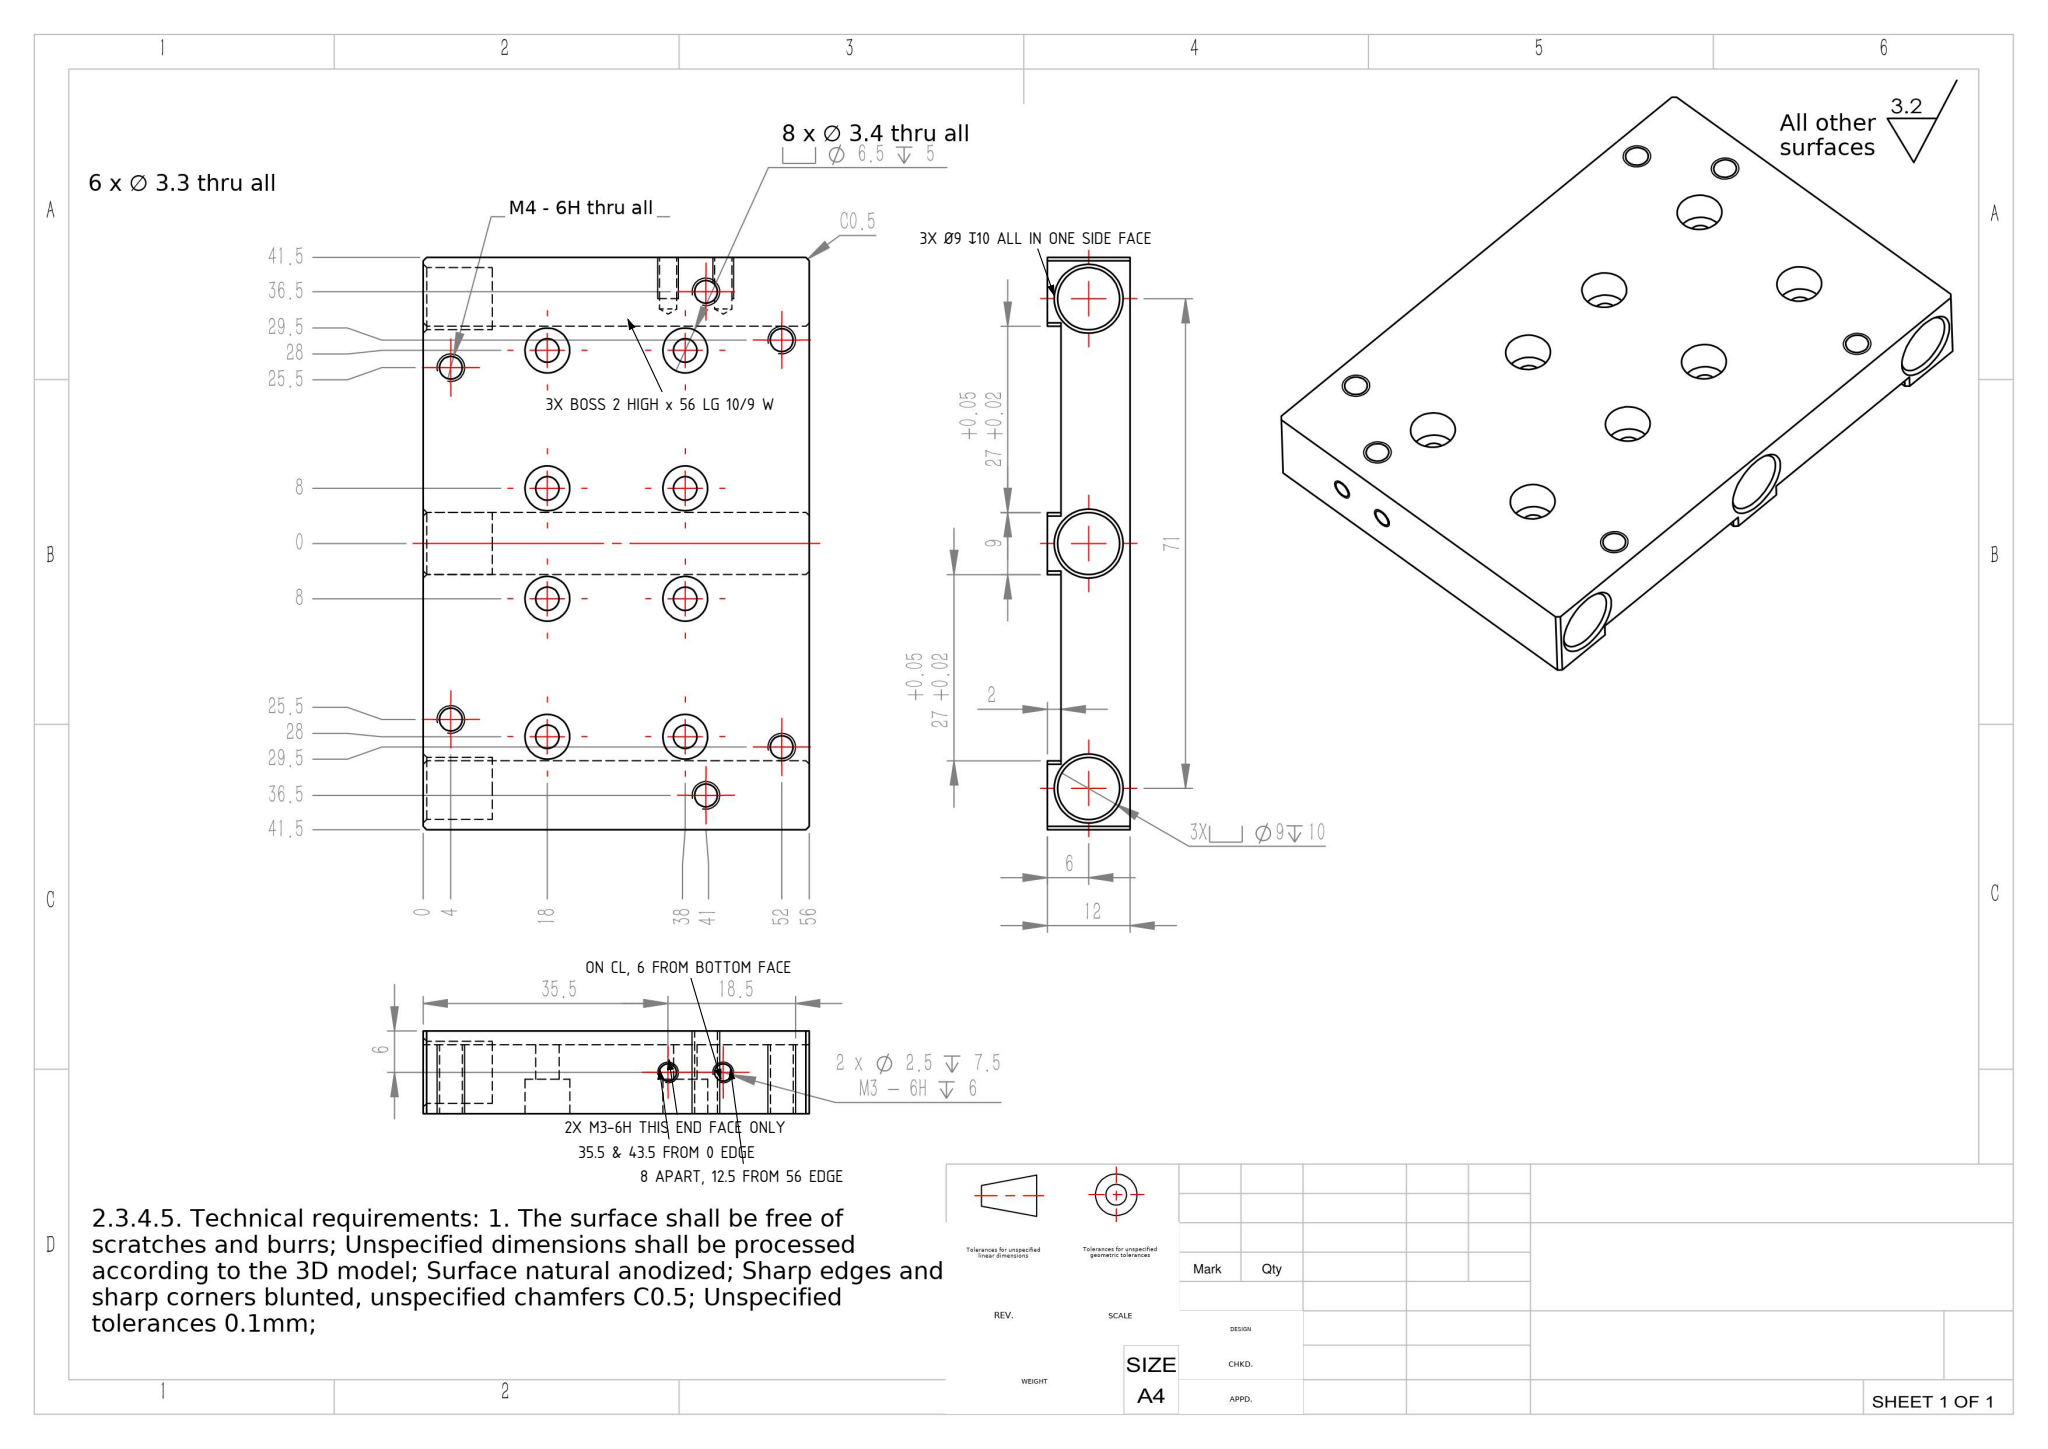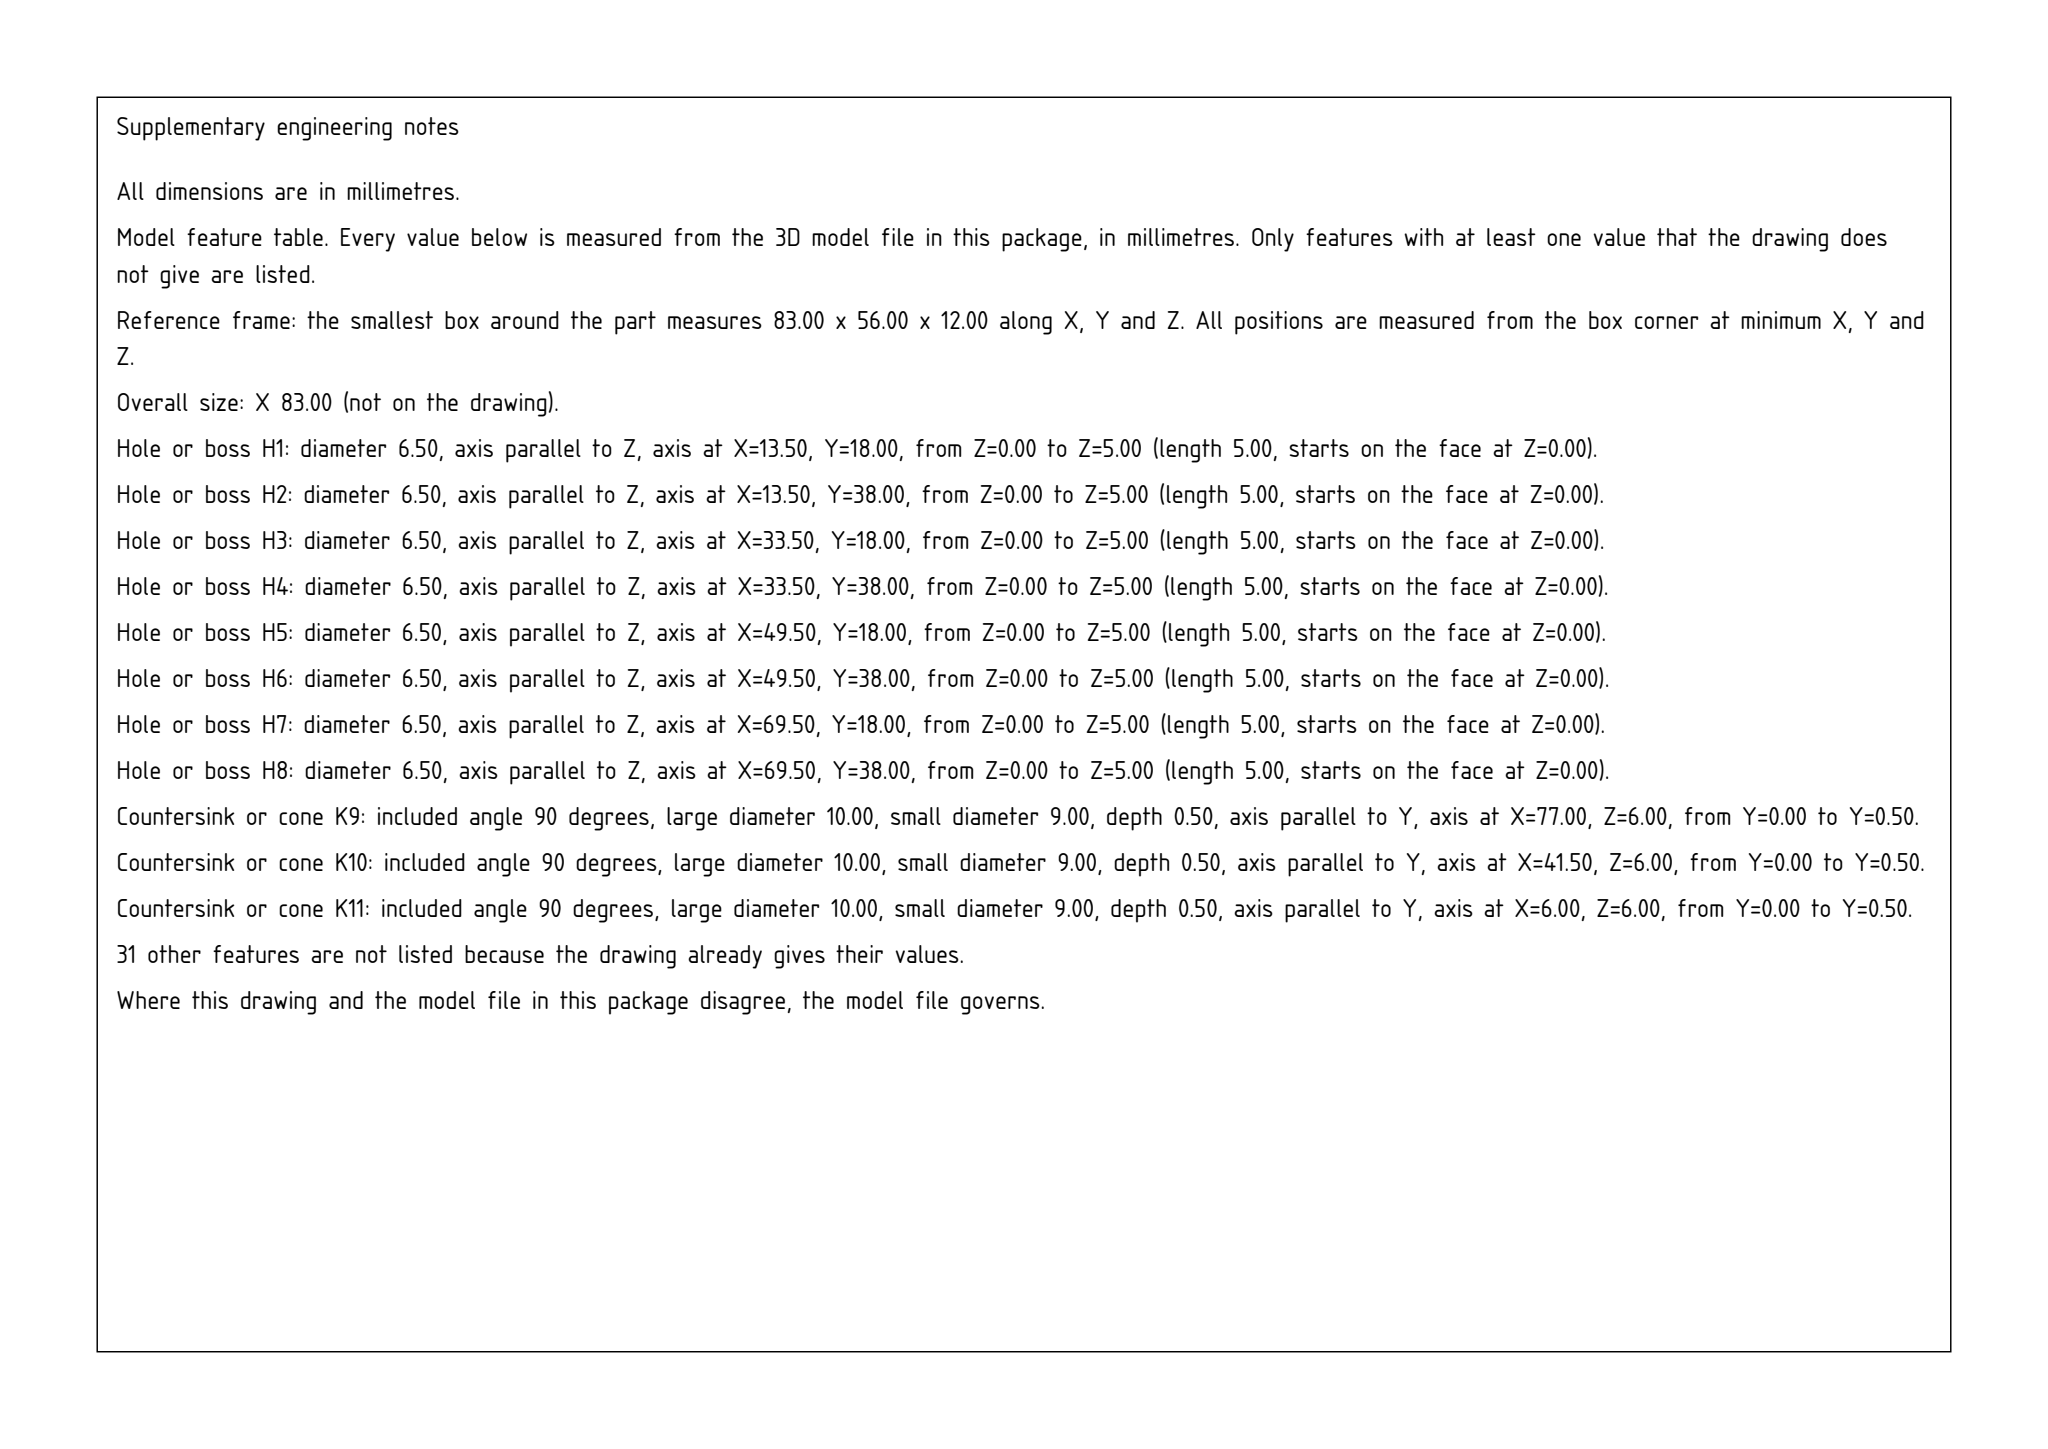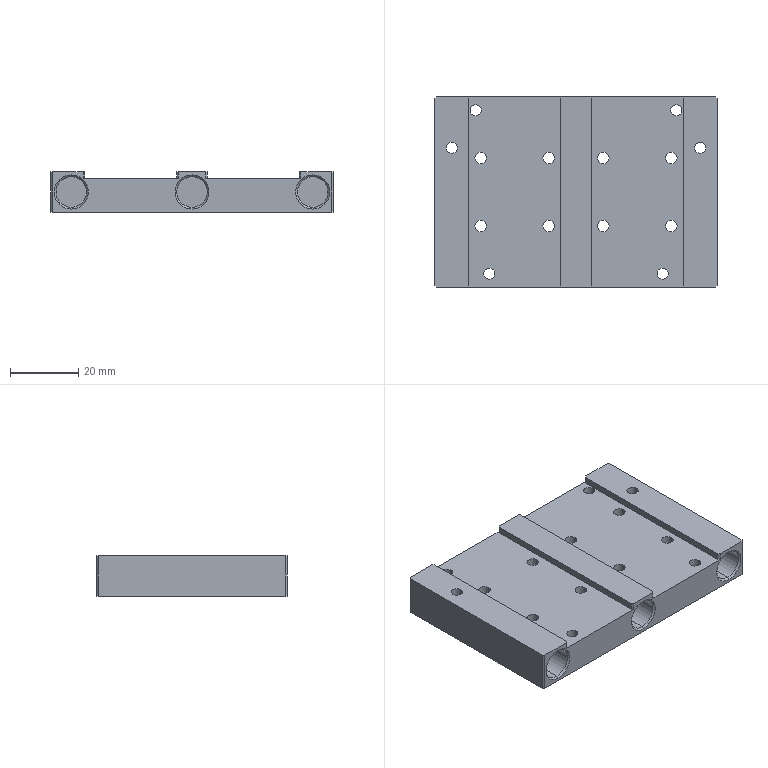Part | SolidWorks | mm | 1 solid | 101 faces | box 83 x 56 x 12 mm | volume 45487 mm3 | cylinder 54 | plane 37 | cone 10 | commonest cylinder face diameters 6.5 x16 3.4 x16 3.3 x12 9 x6 2.5 x4
Drawing notes:
3X BOSS 2 HIGH x 56 LG: 10 WIDE AT EA END, 9 WIDE ON CL | from the solid: z planes 10 (plate top) & 12 (boss tops) -> 2 high; x planes 0/10, 37/46, 73/83; bosses span y 0-56
ALL 3X Ø9 SIDE BORES ENTER THE SAME LONG SIDE FACE (THE 0 EDGE OF THE FRONT VIEW) AT CL 0 AND 35.5 EA SIDE OF CL, CL 6 FROM BOTTOM FACE; NO Ø9 BORE IN EITHER END FACE | from the solid: cylinders Ø9 axis y start at y=0.5 (face y=0, plane y=0 extent x 0.5-82.5, z 0-12) at x=6.0, 41.5, 77.0, z=6.0
2X M3-6H / Ø2.5 HOLES ARE IN THE +41.5 END FACE ONLY; OPPOSITE END FACE (-41.5) IS PLAIN | from the solid: cylinders Ø2.5 axis x from x=75.5 to 83.0 (end face plane x=83.0); no x-axis holes at plane x=0.0
2X M3 END-FACE HOLES AT Y=35.5 & 43.5 FROM BOTTOM EDGE (0) | from the solid: Ø2.5 x-axis holes at (y,z)=(35.5,6.0) and (43.5,6.0), from x=75.5 to 83.0
2X M3 END-FACE HOLES: 8 APART, 12.5 FROM TOP EDGE (56) | from the solid: 43.5-35.5=8; 56.0-43.5=12.5 using bbox y extent 56
2X M3 END-FACE HOLES ON CL, 6 FROM BOTTOM FACE (12 THK) | from the solid: hole axes z=6.0; part thickness z 0-12
build123d program:
from build123d import *

# Parameters (mm, degrees)
SKETCH1_W                                       = 83
SKETCH1_H                                       = 56
BOSS_EXTRUDE1_DEPTH                             = 6
SKETCH2_W                                       = 27
SKETCH2_H                                       = 56
CUT_EXTRUDE1_DEPTH                              = 2
M3_HEX_SOCKET_HEAD_CAP_SCREW_CBORE1_D           = 3.4
M3_HEX_SOCKET_HEAD_CAP_SCREW_CBORE1_CBORE_D     = 6.5
M3_HEX_SOCKET_HEAD_CAP_SCREW_CBORE1_CBORE_DEPTH = 5
SKETCH5_R                                       = 4.5
CUT_EXTRUDE2_DEPTH                              = 10
CHAMFER1_SIZE                                   = 0.5
CHAMFER2_SIZE                                   = 0.5
M4_TAPPED_HOLE1_D                               = 3.3
M3_TAPPED_HOLE1_D                               = 2.5
M3_TAPPED_HOLE1_DEPTH                           = 7.5
M3_TAPPED_HOLE1_TIP                             = 0.7511


with BuildPart() as part:
    # Sketch1 → Boss-Extrude1 (new, symmetric)
    with BuildSketch(Plane.XY):
        Rectangle(SKETCH1_W, SKETCH1_H)
    extrude(amount=BOSS_EXTRUDE1_DEPTH, both=True)

    # Sketch2 → Cut-Extrude1 (cut)
    with BuildSketch(Plane(origin=(0, 0, 6), x_dir=(-1, 0, 0), z_dir=(0, 0, -1))):
        with Locations((-18, 0)):
            Rectangle(SKETCH2_W, SKETCH2_H)
        with Locations((18, 0)):
            Rectangle(SKETCH2_W, SKETCH2_H)
    extrude(amount=CUT_EXTRUDE1_DEPTH, mode=Mode.SUBTRACT)

    # M3 Hex Socket Head Cap Screw CBORE1 (through all)
    with Locations(Plane(origin=(0, 0, -6), x_dir=(-1, 0, 0), z_dir=(0, 0, -1))):
        with Locations((28, 10), (28, -10), (8, -10), (8, 10), (-8, 10), (-8, -10), (-28, -10), (-28, 10)):
            CounterBoreHole(M3_HEX_SOCKET_HEAD_CAP_SCREW_CBORE1_D / 2, M3_HEX_SOCKET_HEAD_CAP_SCREW_CBORE1_CBORE_D / 2, M3_HEX_SOCKET_HEAD_CAP_SCREW_CBORE1_CBORE_DEPTH)

    # Sketch5 → Cut-Extrude2 (cut)
    with BuildSketch(Plane.XZ.offset(28)):
        with Locations(Location((-35.5, 0, 0), (0, 0, 270))):
            Circle(SKETCH5_R)
        with Locations(Location((0, 0, 0), (0, 0, 270))):
            Circle(SKETCH5_R)
        with Locations(Location((35.5, 0, 0), (0, 0, 90))):
            Circle(SKETCH5_R)
    extrude(amount=-CUT_EXTRUDE2_DEPTH, mode=Mode.SUBTRACT)

    # Chamfer1
    chamfer1_edges = [part.edges().sort_by_distance(p)[0] for p in [
        (31.5, 28, 5),
        (31.5, -28, 5),
        (4.5, -28, 5),
        (4.5, 28, 5),
        (-31.5, 28, 5),
        (-4.5, 28, 5),
        (-4.5, -28, 5),
        (-31.5, -28, 5),
        (41.5, -28, 0),
        (-41.5, -28, 0),
        (-41.5, 28, 0),
        (41.5, 28, 0),
    ]]
    chamfer(chamfer1_edges, length=CHAMFER1_SIZE)

    # Chamfer2
    chamfer2_edges = [part.edges().sort_by_distance(p)[0] for p in [
        (-35.5, -28, 4.5),
        (0, -28, 4.5),
        (35.5, -28, -4.5),
    ]]
    chamfer(chamfer2_edges, length=CHAMFER2_SIZE)

    # M4 Tapped Hole1 (through all)
    with Locations(Plane(origin=(0, 0, -6), x_dir=(-1, 0, 0), z_dir=(0, 0, -1))):
        with Locations((36.5, 13), (29.5, 24), (25.5, -24), (-25.5, -24), (-29.5, 24), (-36.5, 13)):
            Hole(M4_TAPPED_HOLE1_D / 2)

    # M3 Tapped Hole1
    with Locations(Plane(origin=(41.5, 0, 0), x_dir=(0, 0, -1), z_dir=(1, 0, 0))):
        with Locations((0, 15.5), (0, 7.5)):
            Hole(M3_TAPPED_HOLE1_D / 2, depth=M3_TAPPED_HOLE1_DEPTH)
            with Locations((0, 0, -(M3_TAPPED_HOLE1_DEPTH + M3_TAPPED_HOLE1_TIP / 2))):  # 118° drill point
                Cone(0, M3_TAPPED_HOLE1_D / 2, M3_TAPPED_HOLE1_TIP, mode=Mode.SUBTRACT)


solid = part.part